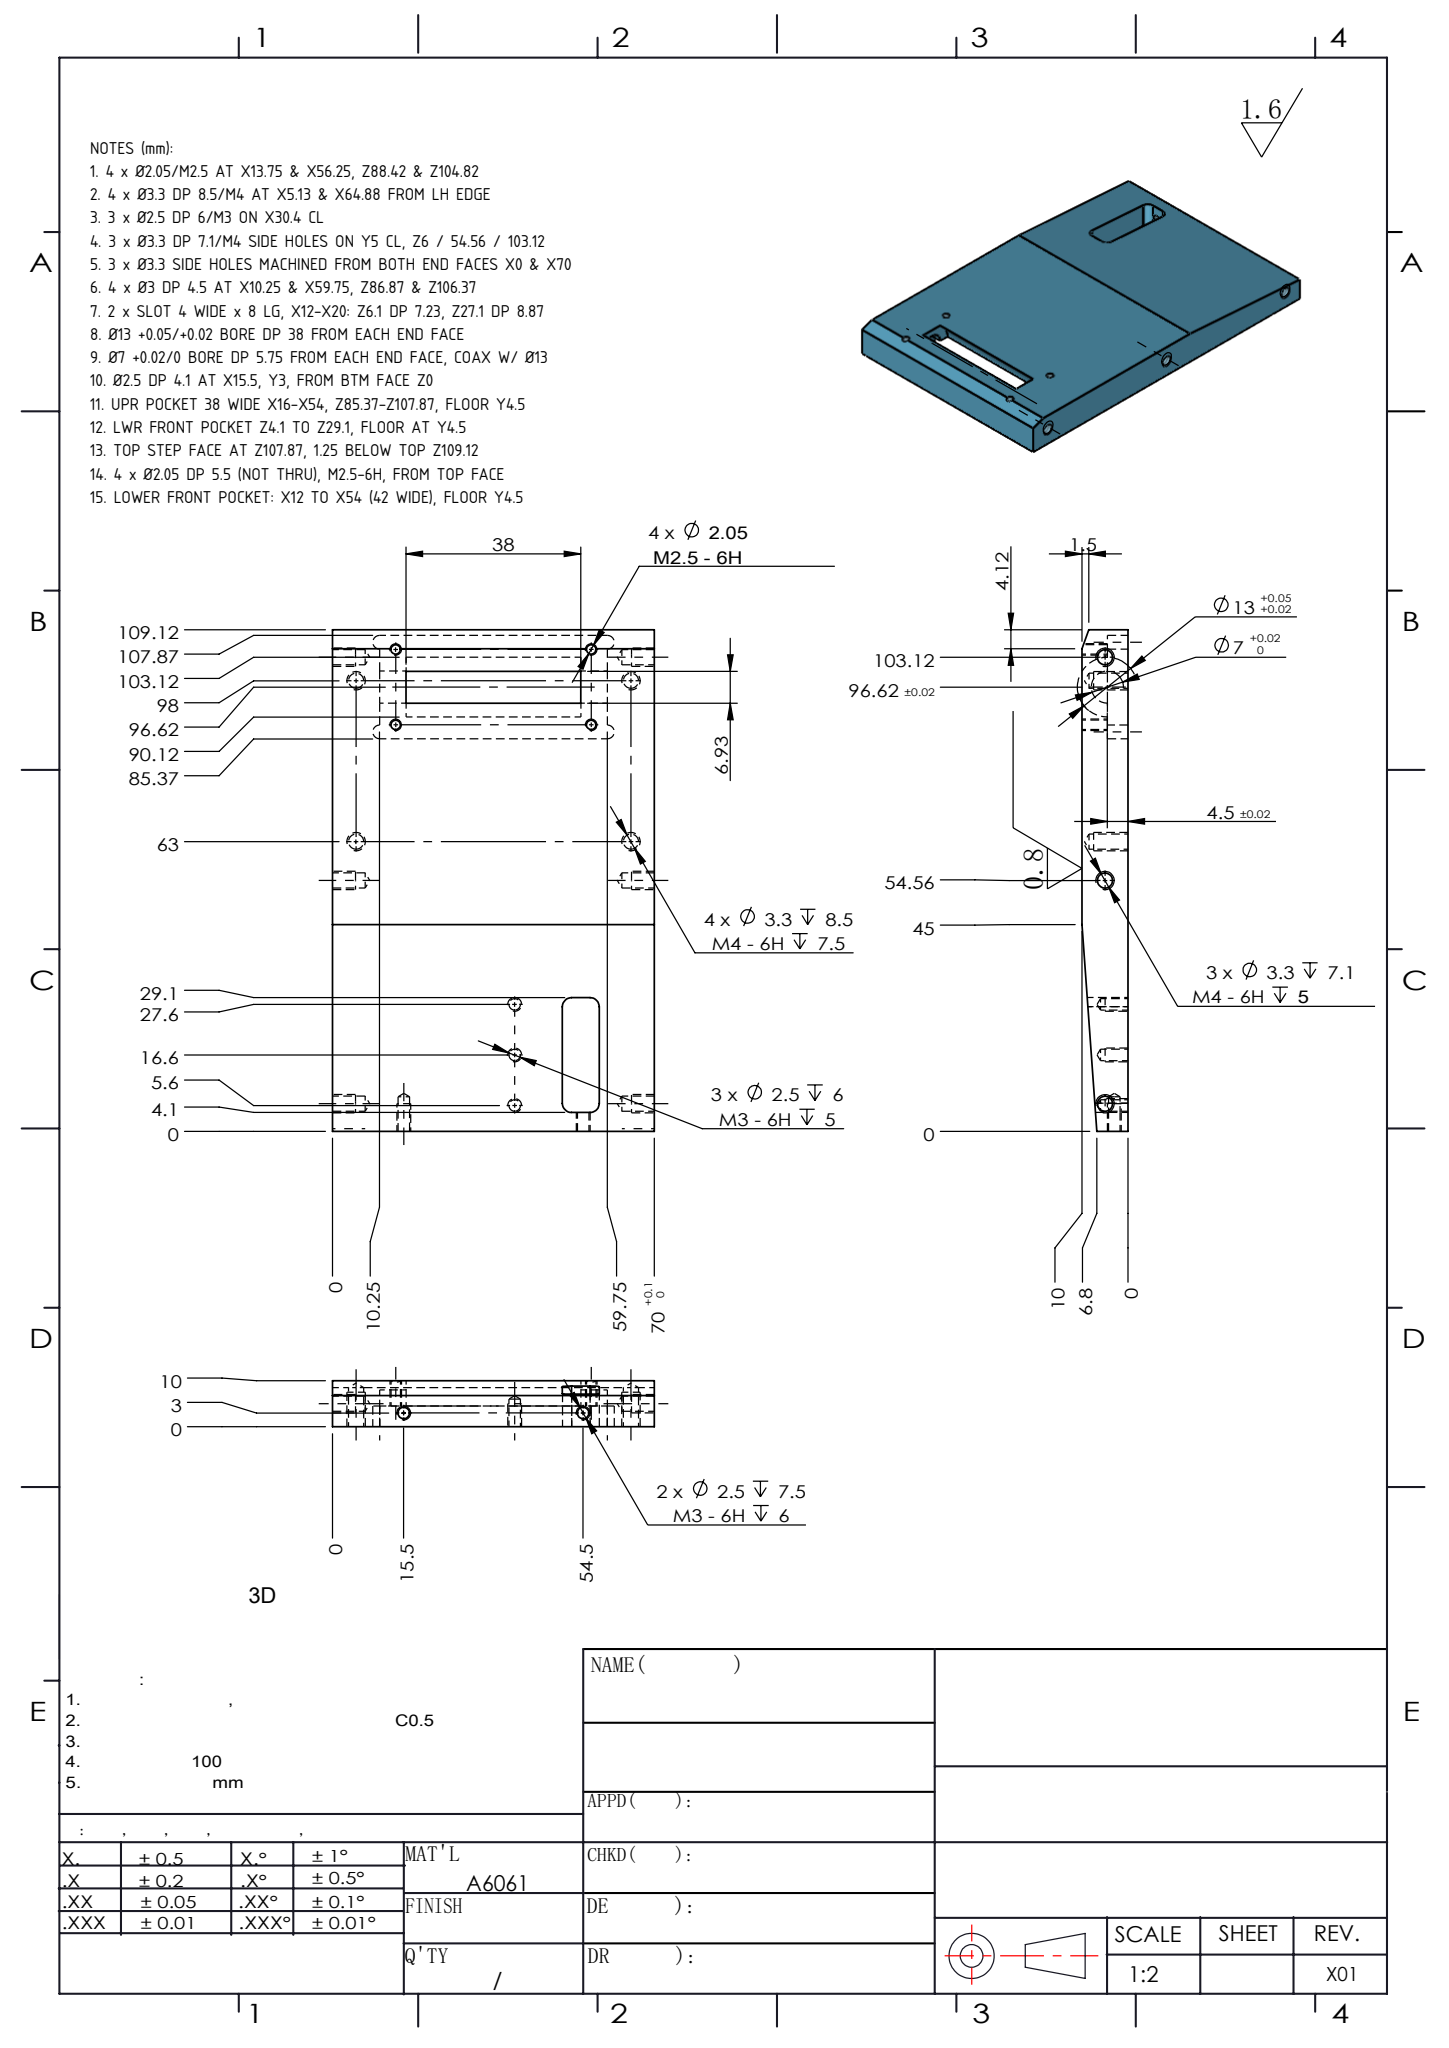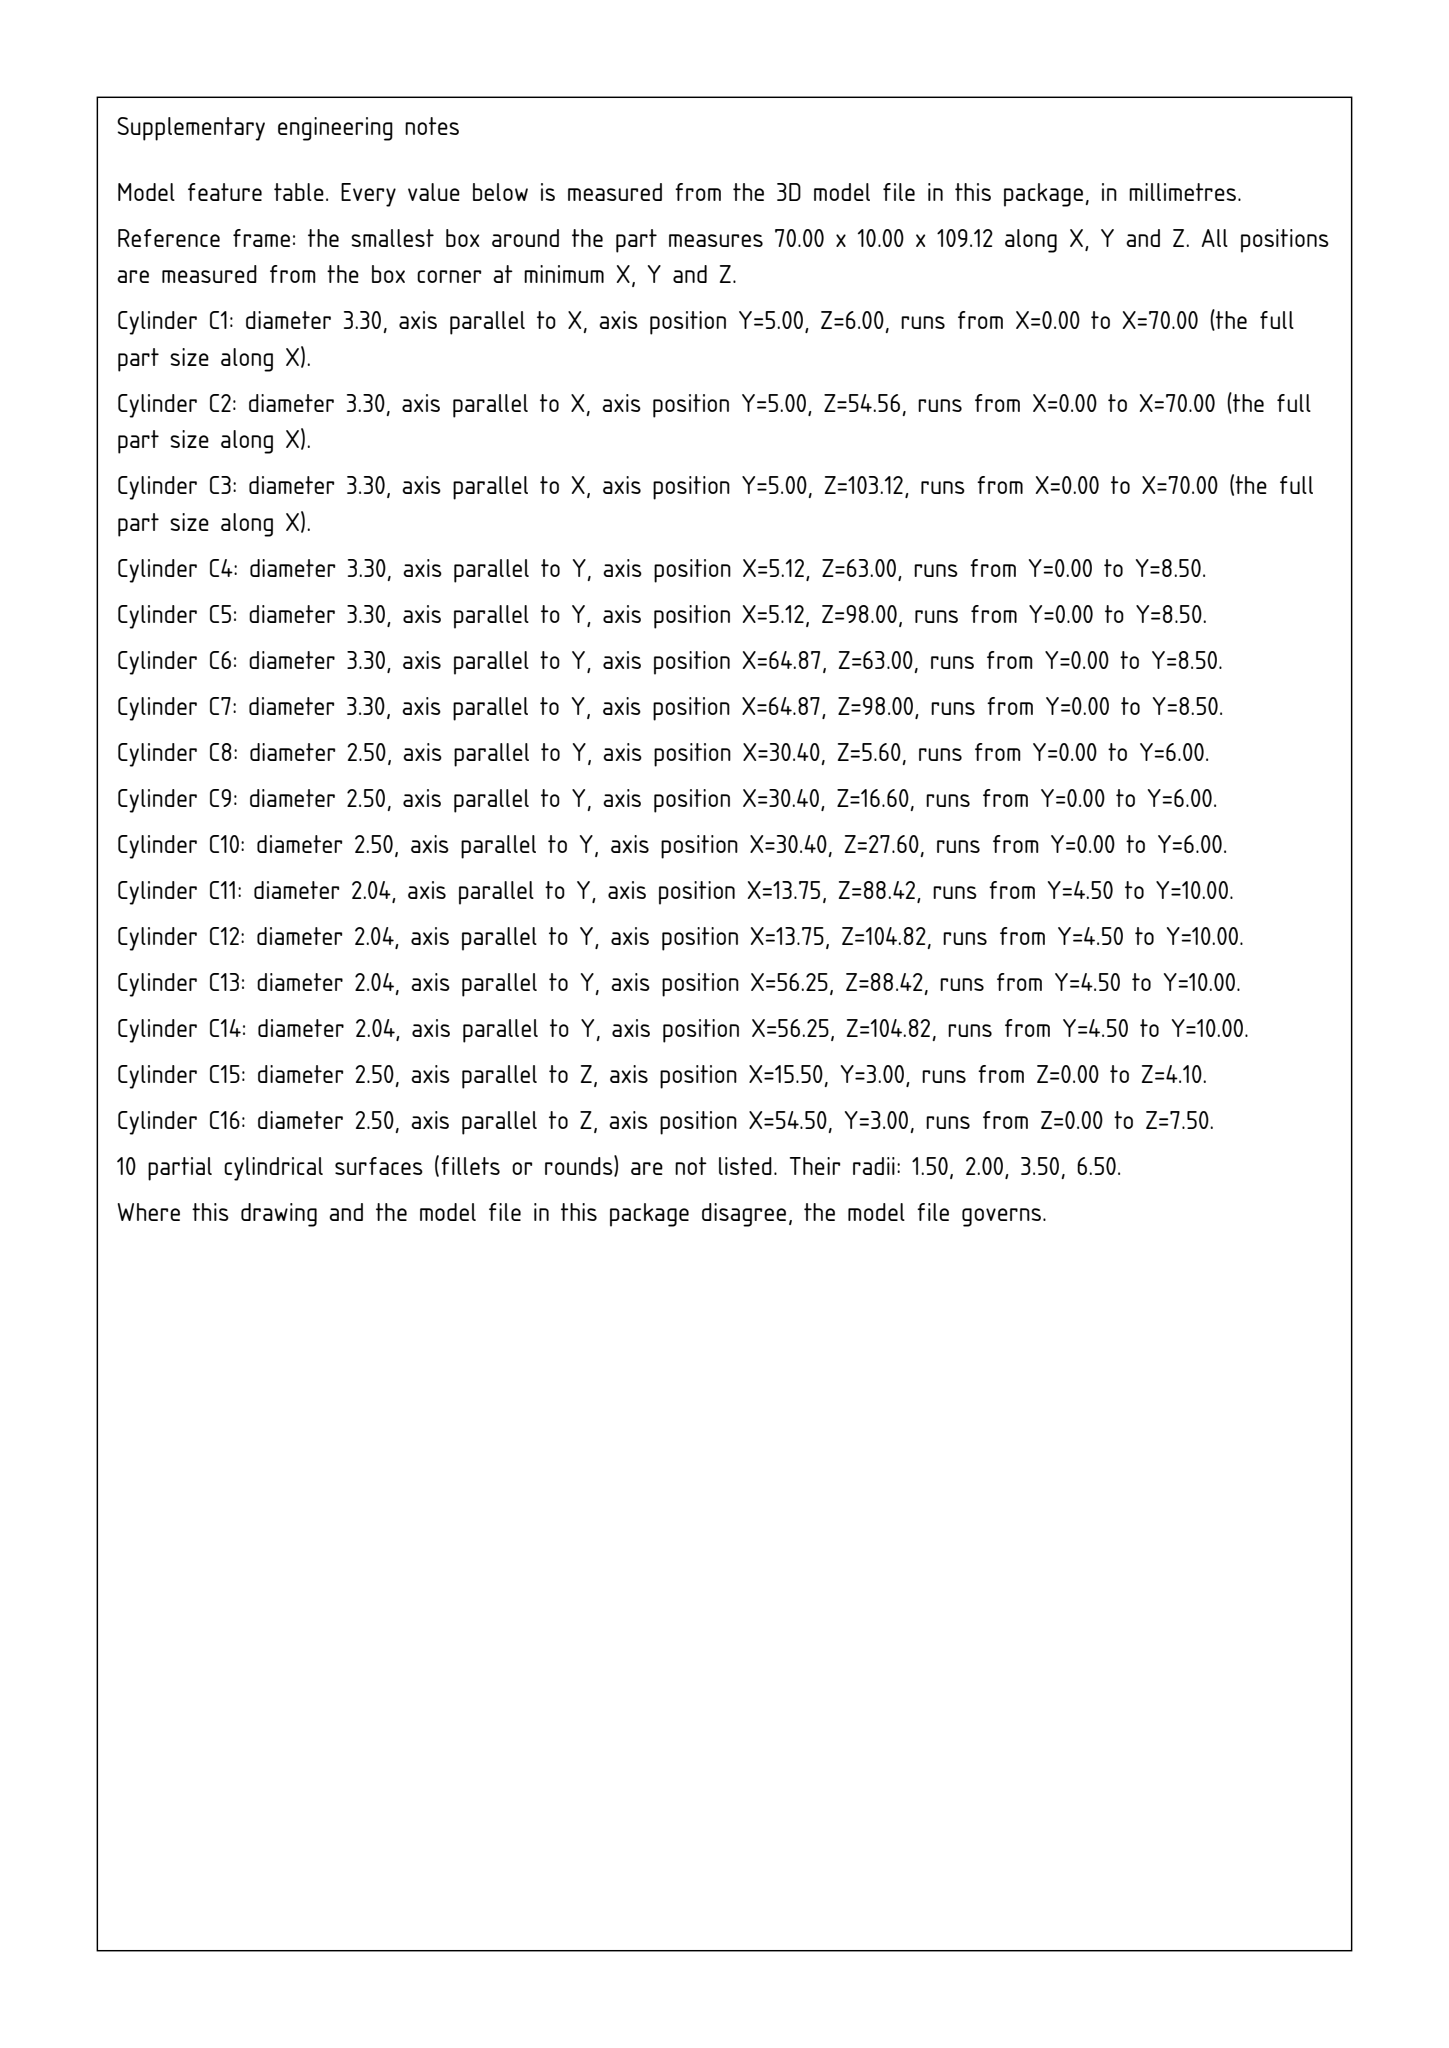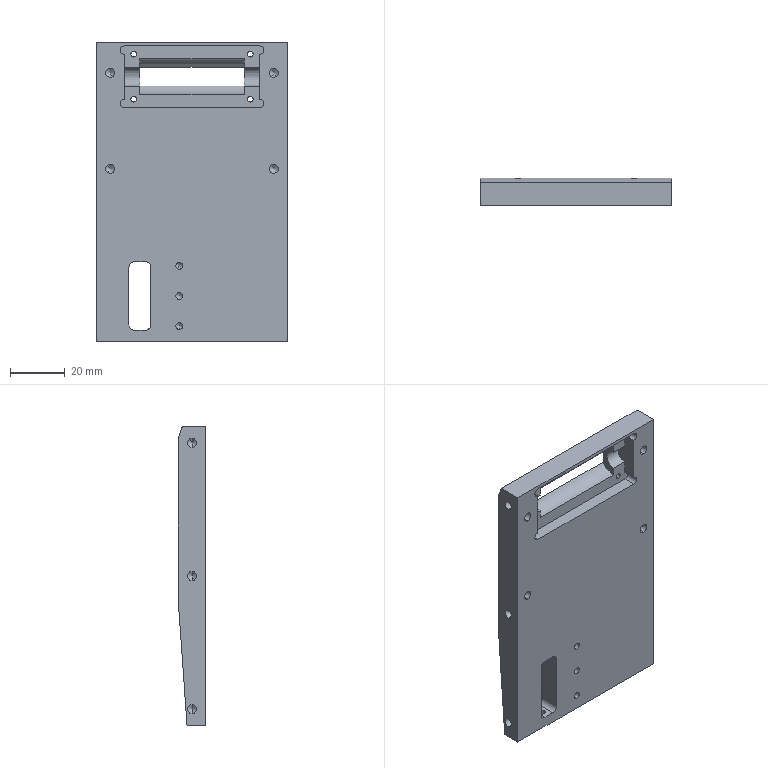Part | SolidWorks | mm | 1 solid | 98 faces | box 70 x 10 x 109.12 mm | volume 61013 mm3 | cylinder 50 | cone 28 | plane 20 | commonest cylinder face diameters 3.3 x20 2.5 x10 2.05 x8 3 x4 4 x4 13 x2 7 x2
Drawing notes:
4 x Ø2.05/M2.5 AT X13.75 & X56.25, Z88.42 & Z104.82 | from the solid: cyl dia2.05 axis y at (13.75/56.25, z 88.42/104.82)
4 x Ø3.3 DP 8.5/M4 AT X5.13 & X64.88 FROM LH EDGE | from the solid: cyl dia3.3 axis y at x5.13/64.88, z63/98, len 8.5
3 x Ø2.5 DP 6/M3 ON X30.4 CL | from the solid: cyl dia2.5 axis y at x30.4, z5.6/16.6/27.6, len 6
3 x Ø3.3 DP 7.1/M4 SIDE HOLES ON Y5 CL, Z6 / 54.56 / 103.12 | from the solid: cyl dia3.3 axis x at y5.0, z6.0/54.56/103.12, len 7.1
3 x Ø3.3 SIDE HOLES MACHINED FROM BOTH END FACES X0 & X70 | from the solid: dia3.3 axis x entries count 4 faces, len 7.1 ea; bbox x 0-70
4 x Ø3 DP 4.5 AT X10.25 & X59.75, Z86.87 & Z106.37 | from the solid: cyl dia3.0 axis y at x10.25/59.75, z86.87/106.37, len 4.5
2 x SLOT 4 WIDE x 8 LG, X12-X20: Z6.1 DP 7.23, Z27.1 DP 8.87 | from the solid: dia4.0 axis y at x14 & x18, z6.1 len7.23 / z27.1 len8.87; planes x12,16,20
Ø13 +0.05/+0.02 BORE DP 38 FROM EACH END FACE | from the solid: cyl dia13 axis x at y4.5 z96.62, len 38, 2 occurrences
Ø7 +0.02/0 BORE DP 5.75 FROM EACH END FACE, COAX W/ Ø13 | from the solid: cyl dia7 axis x at y4.5 z96.62, len 5.75, 2 occurrences
Ø2.5 DP 4.1 AT X15.5, Y3, FROM BTM FACE Z0 | from the solid: cyl dia2.5 axis z at x15.5 y3.0, len 4.1
UPR POCKET 38 WIDE X16-X54, Z85.37-Z107.87, FLOOR Y4.5 | from the solid: planes x16/x54 (38 apart), z85.37/107.87, y4.5
LWR FRONT POCKET Z4.1 TO Z29.1, FLOOR AT Y4.5 | from the solid: planes z4.1, z29.1, y4.5
TOP STEP FACE AT Z107.87, 1.25 BELOW TOP Z109.12 | from the solid: planes z107.87 & z109.12, bbox z 109.12
4 x Ø2.05 DP 5.5 (NOT THRU), M2.5-6H, FROM TOP FACE | from the solid: cylinders Ø2.05 axis y, len 5.5 at x13.75/56.25, z88.42/104.82
LOWER FRONT POCKET: X12 TO X54 (42 WIDE), FLOOR Y4.5 | from the solid: x planes 12.0 & 54.0; y plane 4.5; z4.1-29.1